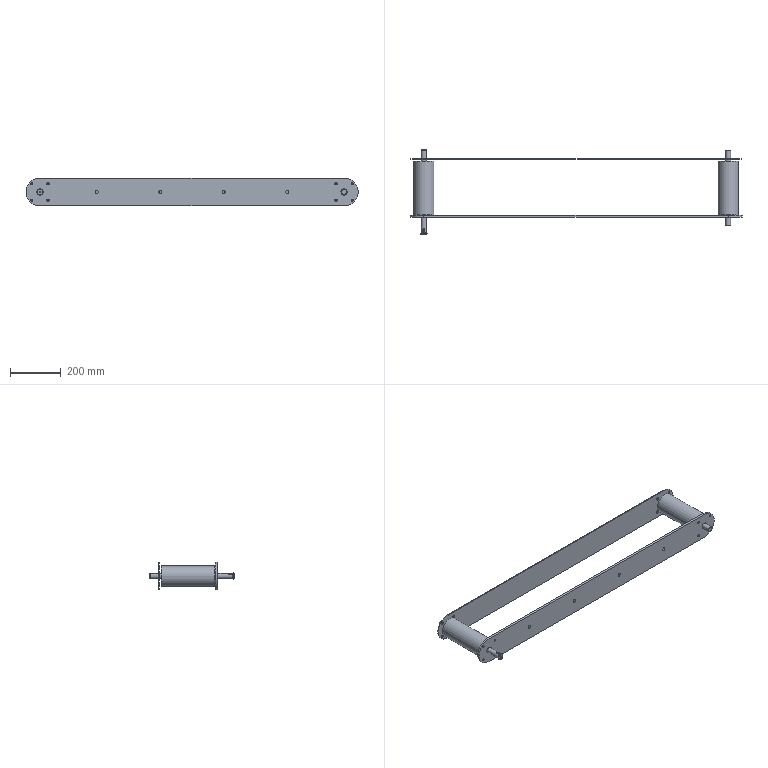Assembly | NX | mm | 6 component files | 6 solids | 75 faces | box 1310 x 331.7 x 110 mm | volume 3394715 mm3 | cylinder 43 | plane 24 | cone 8 | commonest cylinder face diameters 8.5 x8 10 x8 25 x5 110 x4 12 x4 20 x3 4.2 x2 6 x2
Bill of materials:
unnamed part 1 | 1 |  | Long, slender solid round rod with plain flat ends.
unnamed part 2 | 1 |  | Thin, flat, elongated plate with fully rounded ends. Each end has one larger hole with four small holes in a rectangular pattern around it. Four more small holes are evenly spaced along the centerline.
unnamed part 3 | 1 |  | Hollow cylindrical tube or sleeve with a central through-bore. There appears to be a step or counterbore at the bore entrance.
unnamed part 4 | 1 |  | Roller-like body: a large solid cylinder with a smaller coaxial shaft stub at each end. One shaft end has a small center hole and a small slot or notch near its tip.
unnamed part 5 | 1 |  | Stepped circular disc: a larger flange with a smaller concentric raised boss on one face. It has a central through-bore and one small off-center through-hole near the rim. The outer edge on the side away from the boss is chamfered.
unnamed part 6 | 1 |  | Very thin, flat, elongated plate with fully rounded ends. Each end has one larger hole with four small holes in a rectangular pattern around it. There are no holes along the middle span.
Mates:
1. touch align | 131_shaft_2 1 face | 131_roller 1 face
2. touch align | 131_drive_end_roller 1 face | 131_roller 1 face
3. touch align | 131_mount_plate_base 1 face | 131_shaft_2 1 face